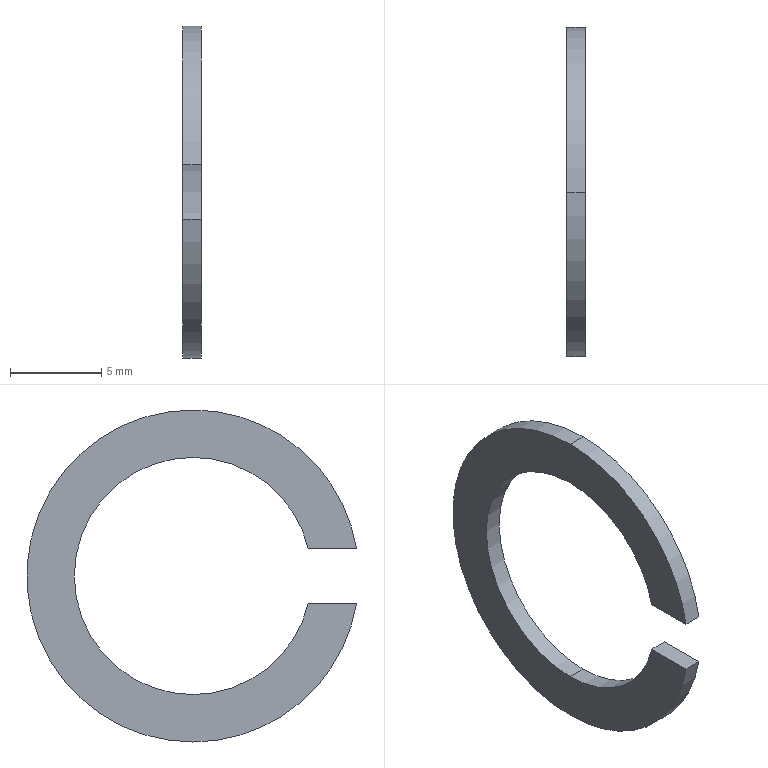Component | SolidWorks | ShaftRetainingRing-15-2 | 1 solid | 10 faces | box 1 x 18.08 x 18.2 mm | volume 120 mm3 | cylinder 6 | plane 4 | commonest cylinder face diameters 18.2 x3 13 x3
build123d program:
from build123d import *

# Parameters (mm, degrees)
BOSS_EXTRUDE1_DEPTH = 1


with BuildPart() as part:
    # Sketch3 → Boss-Extrude1 (new body)
    with BuildSketch(Plane(origin=(0, 0, 0), x_dir=(0, 0, -1), z_dir=(1, 0, 0))):
        with BuildLine():
            Line((1.5, -6.325), (1.5, -8.976))
            ThreePointArc((1.5, -8.976), (0, 9.1), (-1.5, -8.976))
            Line((-1.5, -8.976), (-1.5, -6.325))
            ThreePointArc((-1.5, -6.325), (0, 6.5), (1.5, -6.325))
        make_face()
    extrude(amount=BOSS_EXTRUDE1_DEPTH)


solid = part.part

# Placed as in the assembly
solid = solid.moved(Location((25, 20, 79.212), (0, 0, 0)))
STEP:
#1=COLOUR_RGB('',0.7922,0.8196,0.9333);
#2=FILL_AREA_STYLE_COLOUR('',#1);
#3=FILL_AREA_STYLE('',(#2));
#4=SURFACE_STYLE_FILL_AREA(#3);
#5=SURFACE_SIDE_STYLE('',(#4));
#6=SURFACE_STYLE_USAGE(.BOTH.,#5);
#7=PRESENTATION_STYLE_ASSIGNMENT((#6));
#8=CARTESIAN_POINT('',(1.024,0.7874,2.76));
#9=VERTEX_POINT('',#8);
#10=CARTESIAN_POINT('',(1.024,0.7874,3.477));
#11=VERTEX_POINT('',#10);
#12=CARTESIAN_POINT('',(1.024,0.7874,3.119));
#13=DIRECTION('',(1.,0.,0.));
#14=DIRECTION('',(0.,0.,-1.));
#15=AXIS2_PLACEMENT_3D('',#12,#13,#14);
#16=CIRCLE('',#15,0.3583);
#17=EDGE_CURVE('',#9,#11,#16,.T.);
#18=ORIENTED_EDGE('',*,*,#17,.F.);
#19=CARTESIAN_POINT('',(0.9843,0.7874,2.76));
#20=VERTEX_POINT('',#19);
#21=CARTESIAN_POINT('',(1.024,0.7874,2.76));
#22=DIRECTION('',(-1.,0.,0.));
#23=VECTOR('',#22,39.37);
#24=LINE('',#21,#23);
#25=EDGE_CURVE('',#9,#20,#24,.T.);
#26=ORIENTED_EDGE('',*,*,#25,.T.);
#27=CARTESIAN_POINT('',(0.9843,0.7874,3.477));
#28=VERTEX_POINT('',#27);
#29=CARTESIAN_POINT('',(0.9843,0.7874,3.119));
#30=DIRECTION('',(1.,0.,0.));
#31=DIRECTION('',(0.,0.,-1.));
#32=AXIS2_PLACEMENT_3D('',#29,#30,#31);
#33=CIRCLE('',#32,0.3583);
#34=EDGE_CURVE('',#20,#28,#33,.T.);
#35=ORIENTED_EDGE('',*,*,#34,.T.);
#36=CARTESIAN_POINT('',(1.024,0.7874,3.477));
#37=DIRECTION('',(-1.,0.,0.));
#38=VECTOR('',#37,39.37);
#39=LINE('',#36,#38);
#40=EDGE_CURVE('',#11,#28,#39,.T.);
#41=ORIENTED_EDGE('',*,*,#40,.F.);
#42=EDGE_LOOP('',(#18,#26,#35,#41));
#43=FACE_OUTER_BOUND('',#42,.T.);
#44=CARTESIAN_POINT('',(1.024,0.7874,3.119));
#45=DIRECTION('',(-1.,0.,0.));
#46=DIRECTION('',(0.,0.,1.));
#47=AXIS2_PLACEMENT_3D('',#44,#45,#46);
#48=CYLINDRICAL_SURFACE('',#47,0.3583);
#49=ADVANCED_FACE('',(#43),#48,.T.);
#50=CARTESIAN_POINT('',(1.024,0.434,3.178));
#51=VERTEX_POINT('',#50);
#52=CARTESIAN_POINT('',(1.024,0.7874,3.119));
#53=DIRECTION('',(1.,0.,0.));
#54=DIRECTION('',(0.,0.,-1.));
#55=AXIS2_PLACEMENT_3D('',#52,#53,#54);
#56=CIRCLE('',#55,0.3583);
#57=EDGE_CURVE('',#11,#51,#56,.T.);
#58=ORIENTED_EDGE('',*,*,#57,.F.);
#59=ORIENTED_EDGE('',*,*,#40,.T.);
#60=CARTESIAN_POINT('',(0.9843,0.434,3.178));
#61=VERTEX_POINT('',#60);
#62=CARTESIAN_POINT('',(0.9843,0.7874,3.119));
#63=DIRECTION('',(1.,0.,0.));
#64=DIRECTION('',(0.,0.,-1.));
#65=AXIS2_PLACEMENT_3D('',#62,#63,#64);
#66=CIRCLE('',#65,0.3583);
#67=EDGE_CURVE('',#28,#61,#66,.T.);
#68=ORIENTED_EDGE('',*,*,#67,.T.);
#69=CARTESIAN_POINT('',(1.024,0.434,3.178));
#70=DIRECTION('',(-1.,0.,0.));
#71=VECTOR('',#70,39.37);
#72=LINE('',#69,#71);
#73=EDGE_CURVE('',#51,#61,#72,.T.);
#74=ORIENTED_EDGE('',*,*,#73,.F.);
#75=EDGE_LOOP('',(#58,#59,#68,#74));
#76=FACE_OUTER_BOUND('',#75,.T.);
#77=CARTESIAN_POINT('',(1.024,0.7874,3.119));
#78=DIRECTION('',(-1.,0.,0.));
#79=DIRECTION('',(0.,0.,1.));
#80=AXIS2_PLACEMENT_3D('',#77,#78,#79);
#81=CYLINDRICAL_SURFACE('',#80,0.3583);
#82=ADVANCED_FACE('',(#76),#81,.T.);
#83=CARTESIAN_POINT('',(1.024,0.7874,2.863));
#84=VERTEX_POINT('',#83);
#85=CARTESIAN_POINT('',(1.024,0.5384,3.06));
#86=VERTEX_POINT('',#85);
#87=CARTESIAN_POINT('',(1.024,0.7874,3.119));
#88=DIRECTION('',(-1.,0.,0.));
#89=DIRECTION('',(0.,0.,-1.));
#90=AXIS2_PLACEMENT_3D('',#87,#88,#89);
#91=CIRCLE('',#90,0.2559);
#92=EDGE_CURVE('',#84,#86,#91,.T.);
#93=ORIENTED_EDGE('',*,*,#92,.F.);
#94=CARTESIAN_POINT('',(0.9843,0.7874,2.863));
#95=VERTEX_POINT('',#94);
#96=CARTESIAN_POINT('',(1.024,0.7874,2.863));
#97=DIRECTION('',(-1.,0.,0.));
#98=VECTOR('',#97,39.37);
#99=LINE('',#96,#98);
#100=EDGE_CURVE('',#84,#95,#99,.T.);
#101=ORIENTED_EDGE('',*,*,#100,.T.);
#102=CARTESIAN_POINT('',(0.9843,0.5384,3.06));
#103=VERTEX_POINT('',#102);
#104=CARTESIAN_POINT('',(0.9843,0.7874,3.119));
#105=DIRECTION('',(-1.,0.,0.));
#106=DIRECTION('',(0.,0.,-1.));
#107=AXIS2_PLACEMENT_3D('',#104,#105,#106);
#108=CIRCLE('',#107,0.2559);
#109=EDGE_CURVE('',#95,#103,#108,.T.);
#110=ORIENTED_EDGE('',*,*,#109,.T.);
#111=CARTESIAN_POINT('',(1.024,0.5384,3.06));
#112=DIRECTION('',(-1.,0.,0.));
#113=VECTOR('',#112,39.37);
#114=LINE('',#111,#113);
#115=EDGE_CURVE('',#86,#103,#114,.T.);
#116=ORIENTED_EDGE('',*,*,#115,.F.);
#117=EDGE_LOOP('',(#93,#101,#110,#116));
#118=FACE_OUTER_BOUND('',#117,.T.);
#119=CARTESIAN_POINT('',(1.024,0.7874,3.119));
#120=DIRECTION('',(-1.,0.,0.));
#121=DIRECTION('',(0.,0.,1.));
#122=AXIS2_PLACEMENT_3D('',#119,#120,#121);
#123=CYLINDRICAL_SURFACE('',#122,0.2559);
#124=ADVANCED_FACE('',(#118),#123,.F.);
#125=ORIENTED_EDGE('',*,*,#100,.F.);
#126=CARTESIAN_POINT('',(1.024,0.7874,3.375));
#127=VERTEX_POINT('',#126);
#128=CARTESIAN_POINT('',(1.024,0.7874,3.119));
#129=DIRECTION('',(-1.,0.,0.));
#130=DIRECTION('',(0.,0.,-1.));
#131=AXIS2_PLACEMENT_3D('',#128,#129,#130);
#132=CIRCLE('',#131,0.2559);
#133=EDGE_CURVE('',#127,#84,#132,.T.);
#134=ORIENTED_EDGE('',*,*,#133,.F.);
#135=CARTESIAN_POINT('',(0.9843,0.7874,3.375));
#136=VERTEX_POINT('',#135);
#137=CARTESIAN_POINT('',(1.024,0.7874,3.375));
#138=DIRECTION('',(-1.,0.,0.));
#139=VECTOR('',#138,39.37);
#140=LINE('',#137,#139);
#141=EDGE_CURVE('',#127,#136,#140,.T.);
#142=ORIENTED_EDGE('',*,*,#141,.T.);
#143=CARTESIAN_POINT('',(0.9843,0.7874,3.119));
#144=DIRECTION('',(-1.,0.,0.));
#145=DIRECTION('',(0.,0.,-1.));
#146=AXIS2_PLACEMENT_3D('',#143,#144,#145);
#147=CIRCLE('',#146,0.2559);
#148=EDGE_CURVE('',#136,#95,#147,.T.);
#149=ORIENTED_EDGE('',*,*,#148,.T.);
#150=EDGE_LOOP('',(#125,#134,#142,#149));
#151=FACE_OUTER_BOUND('',#150,.T.);
#152=CARTESIAN_POINT('',(1.024,0.7874,3.119));
#153=DIRECTION('',(-1.,0.,0.));
#154=DIRECTION('',(0.,0.,1.));
#155=AXIS2_PLACEMENT_3D('',#152,#153,#154);
#156=CYLINDRICAL_SURFACE('',#155,0.2559);
#157=ADVANCED_FACE('',(#151),#156,.F.);
#158=ORIENTED_EDGE('',*,*,#141,.F.);
#159=CARTESIAN_POINT('',(1.024,0.5384,3.178));
#160=VERTEX_POINT('',#159);
#161=CARTESIAN_POINT('',(1.024,0.7874,3.119));
#162=DIRECTION('',(-1.,0.,0.));
#163=DIRECTION('',(0.,0.,-1.));
#164=AXIS2_PLACEMENT_3D('',#161,#162,#163);
#165=CIRCLE('',#164,0.2559);
#166=EDGE_CURVE('',#160,#127,#165,.T.);
#167=ORIENTED_EDGE('',*,*,#166,.F.);
#168=CARTESIAN_POINT('',(0.9843,0.5384,3.178));
#169=VERTEX_POINT('',#168);
#170=CARTESIAN_POINT('',(1.024,0.5384,3.178));
#171=DIRECTION('',(-1.,0.,0.));
#172=VECTOR('',#171,39.37);
#173=LINE('',#170,#172);
#174=EDGE_CURVE('',#160,#169,#173,.T.);
#175=ORIENTED_EDGE('',*,*,#174,.T.);
#176=CARTESIAN_POINT('',(0.9843,0.7874,3.119));
#177=DIRECTION('',(-1.,0.,0.));
#178=DIRECTION('',(0.,0.,-1.));
#179=AXIS2_PLACEMENT_3D('',#176,#177,#178);
#180=CIRCLE('',#179,0.2559);
#181=EDGE_CURVE('',#169,#136,#180,.T.);
#182=ORIENTED_EDGE('',*,*,#181,.T.);
#183=EDGE_LOOP('',(#158,#167,#175,#182));
#184=FACE_OUTER_BOUND('',#183,.T.);
#185=CARTESIAN_POINT('',(1.024,0.7874,3.119));
#186=DIRECTION('',(-1.,0.,0.));
#187=DIRECTION('',(0.,0.,1.));
#188=AXIS2_PLACEMENT_3D('',#185,#186,#187);
#189=CYLINDRICAL_SURFACE('',#188,0.2559);
#190=ADVANCED_FACE('',(#184),#189,.F.);
#191=CARTESIAN_POINT('',(0.9843,0.434,3.06));
#192=VERTEX_POINT('',#191);
#193=CARTESIAN_POINT('',(0.9843,0.5384,3.06));
#194=DIRECTION('',(0.,-1.,0.));
#195=VECTOR('',#194,39.37);
#196=LINE('',#193,#195);
#197=EDGE_CURVE('',#103,#192,#196,.T.);
#198=ORIENTED_EDGE('',*,*,#197,.T.);
#199=CARTESIAN_POINT('',(1.024,0.434,3.06));
#200=VERTEX_POINT('',#199);
#201=CARTESIAN_POINT('',(1.024,0.434,3.06));
#202=DIRECTION('',(-1.,0.,0.));
#203=VECTOR('',#202,39.37);
#204=LINE('',#201,#203);
#205=EDGE_CURVE('',#200,#192,#204,.T.);
#206=ORIENTED_EDGE('',*,*,#205,.F.);
#207=CARTESIAN_POINT('',(1.024,0.5384,3.06));
#208=DIRECTION('',(0.,-1.,0.));
#209=VECTOR('',#208,39.37);
#210=LINE('',#207,#209);
#211=EDGE_CURVE('',#86,#200,#210,.T.);
#212=ORIENTED_EDGE('',*,*,#211,.F.);
#213=ORIENTED_EDGE('',*,*,#115,.T.);
#214=EDGE_LOOP('',(#198,#206,#212,#213));
#215=FACE_OUTER_BOUND('',#214,.T.);
#216=CARTESIAN_POINT('',(1.024,0.5384,3.06));
#217=DIRECTION('',(0.,0.,-1.));
#218=DIRECTION('',(-1.,0.,0.));
#219=AXIS2_PLACEMENT_3D('',#216,#217,#218);
#220=PLANE('',#219);
#221=ADVANCED_FACE('',(#215),#220,.F.);
#222=ORIENTED_EDGE('',*,*,#25,.F.);
#223=CARTESIAN_POINT('',(1.024,0.7874,3.119));
#224=DIRECTION('',(1.,0.,0.));
#225=DIRECTION('',(0.,0.,-1.));
#226=AXIS2_PLACEMENT_3D('',#223,#224,#225);
#227=CIRCLE('',#226,0.3583);
#228=EDGE_CURVE('',#200,#9,#227,.T.);
#229=ORIENTED_EDGE('',*,*,#228,.F.);
#230=ORIENTED_EDGE('',*,*,#205,.T.);
#231=CARTESIAN_POINT('',(0.9843,0.7874,3.119));
#232=DIRECTION('',(1.,0.,0.));
#233=DIRECTION('',(0.,0.,-1.));
#234=AXIS2_PLACEMENT_3D('',#231,#232,#233);
#235=CIRCLE('',#234,0.3583);
#236=EDGE_CURVE('',#192,#20,#235,.T.);
#237=ORIENTED_EDGE('',*,*,#236,.T.);
#238=EDGE_LOOP('',(#222,#229,#230,#237));
#239=FACE_OUTER_BOUND('',#238,.T.);
#240=CARTESIAN_POINT('',(1.024,0.7874,3.119));
#241=DIRECTION('',(-1.,0.,0.));
#242=DIRECTION('',(0.,0.,1.));
#243=AXIS2_PLACEMENT_3D('',#240,#241,#242);
#244=CYLINDRICAL_SURFACE('',#243,0.3583);
#245=ADVANCED_FACE('',(#239),#244,.T.);
#246=CARTESIAN_POINT('',(0.9843,0.5384,3.178));
#247=DIRECTION('',(0.,1.,0.));
#248=VECTOR('',#247,39.37);
#249=LINE('',#246,#248);
#250=EDGE_CURVE('',#61,#169,#249,.T.);
#251=ORIENTED_EDGE('',*,*,#250,.T.);
#252=ORIENTED_EDGE('',*,*,#174,.F.);
#253=CARTESIAN_POINT('',(1.024,0.5384,3.178));
#254=DIRECTION('',(0.,1.,0.));
#255=VECTOR('',#254,39.37);
#256=LINE('',#253,#255);
#257=EDGE_CURVE('',#51,#160,#256,.T.);
#258=ORIENTED_EDGE('',*,*,#257,.F.);
#259=ORIENTED_EDGE('',*,*,#73,.T.);
#260=EDGE_LOOP('',(#251,#252,#258,#259));
#261=FACE_OUTER_BOUND('',#260,.T.);
#262=CARTESIAN_POINT('',(1.024,0.5384,3.178));
#263=DIRECTION('',(0.,0.,1.));
#264=DIRECTION('',(1.,0.,0.));
#265=AXIS2_PLACEMENT_3D('',#262,#263,#264);
#266=PLANE('',#265);
#267=ADVANCED_FACE('',(#261),#266,.F.);
#268=ORIENTED_EDGE('',*,*,#166,.T.);
#269=ORIENTED_EDGE('',*,*,#133,.T.);
#270=ORIENTED_EDGE('',*,*,#92,.T.);
#271=ORIENTED_EDGE('',*,*,#211,.T.);
#272=ORIENTED_EDGE('',*,*,#228,.T.);
#273=ORIENTED_EDGE('',*,*,#17,.T.);
#274=ORIENTED_EDGE('',*,*,#57,.T.);
#275=ORIENTED_EDGE('',*,*,#257,.T.);
#276=EDGE_LOOP('',(#268,#269,#270,#271,#272,#273,#274,#275));
#277=FACE_OUTER_BOUND('',#276,.T.);
#278=CARTESIAN_POINT('',(1.024,0.7874,3.119));
#279=DIRECTION('',(1.,0.,0.));
#280=DIRECTION('',(0.,0.,-1.));
#281=AXIS2_PLACEMENT_3D('',#278,#279,#280);
#282=PLANE('',#281);
#283=ADVANCED_FACE('',(#277),#282,.T.);
#284=ORIENTED_EDGE('',*,*,#181,.F.);
#285=ORIENTED_EDGE('',*,*,#250,.F.);
#286=ORIENTED_EDGE('',*,*,#67,.F.);
#287=ORIENTED_EDGE('',*,*,#34,.F.);
#288=ORIENTED_EDGE('',*,*,#236,.F.);
#289=ORIENTED_EDGE('',*,*,#197,.F.);
#290=ORIENTED_EDGE('',*,*,#109,.F.);
#291=ORIENTED_EDGE('',*,*,#148,.F.);
#292=EDGE_LOOP('',(#284,#285,#286,#287,#288,#289,#290,#291));
#293=FACE_OUTER_BOUND('',#292,.T.);
#294=CARTESIAN_POINT('',(0.9843,0.7874,3.119));
#295=DIRECTION('',(1.,0.,0.));
#296=DIRECTION('',(0.,0.,-1.));
#297=AXIS2_PLACEMENT_3D('',#294,#295,#296);
#298=PLANE('',#297);
#299=ADVANCED_FACE('',(#293),#298,.F.);
#300=CLOSED_SHELL('',(#49,#82,#124,#157,#190,#221,#245,#267,#283,#299));
#301=MANIFOLD_SOLID_BREP('',#300);
#302=STYLED_ITEM('',(#7),#301);
#303=PRESENTATION_LAYER_ASSIGNMENT('','',(#302));
#304=CARTESIAN_POINT('',(0.,0.,0.));
#305=DIRECTION('',(0.,0.,1.));
#306=DIRECTION('',(1.,0.,0.));
#307=AXIS2_PLACEMENT_3D('',#304,#305,#306);
#308=(LENGTH_UNIT()NAMED_UNIT(*)SI_UNIT($,.METRE.));
#309=LENGTH_MEASURE_WITH_UNIT(LENGTH_MEASURE(0.0254),#308);
#310=DIMENSIONAL_EXPONENTS(1.,0.,0.,0.,0.,0.,0.);
#311=(CONVERSION_BASED_UNIT('',#309)LENGTH_UNIT()NAMED_UNIT(#310));
#312=UNCERTAINTY_MEASURE_WITH_UNIT(LENGTH_MEASURE(0.00001),#311,'','');
#313=(NAMED_UNIT(*)PLANE_ANGLE_UNIT()SI_UNIT($,.RADIAN.));
#314=(NAMED_UNIT(*)SI_UNIT($,.STERADIAN.)SOLID_ANGLE_UNIT());
#315=(GEOMETRIC_REPRESENTATION_CONTEXT(3)GLOBAL_UNCERTAINTY_ASSIGNED_CONTEXT((#312))GLOBAL_UNIT_ASSIGNED_CONTEXT((#311,#313,#314))REPRESENTATION_CONTEXT('',''));
#316=ADVANCED_BREP_SHAPE_REPRESENTATION('',(#301,#307),#315);
#317=(LENGTH_UNIT()NAMED_UNIT(*)SI_UNIT($,.METRE.));
#318=LENGTH_MEASURE_WITH_UNIT(LENGTH_MEASURE(0.0254),#317);
#319=DIMENSIONAL_EXPONENTS(1.,0.,0.,0.,0.,0.,0.);
#320=(CONVERSION_BASED_UNIT('',#318)LENGTH_UNIT()NAMED_UNIT(#319));
#321=UNCERTAINTY_MEASURE_WITH_UNIT(LENGTH_MEASURE(0.00001),#320,'','');
#322=(NAMED_UNIT(*)PLANE_ANGLE_UNIT()SI_UNIT($,.RADIAN.));
#323=(NAMED_UNIT(*)SI_UNIT($,.STERADIAN.)SOLID_ANGLE_UNIT());
#324=(GEOMETRIC_REPRESENTATION_CONTEXT(3)GLOBAL_UNCERTAINTY_ASSIGNED_CONTEXT((#321))GLOBAL_UNIT_ASSIGNED_CONTEXT((#320,#322,#323))REPRESENTATION_CONTEXT('',''));
#325=MECHANICAL_DESIGN_GEOMETRIC_PRESENTATION_REPRESENTATION('',(#302),#324);